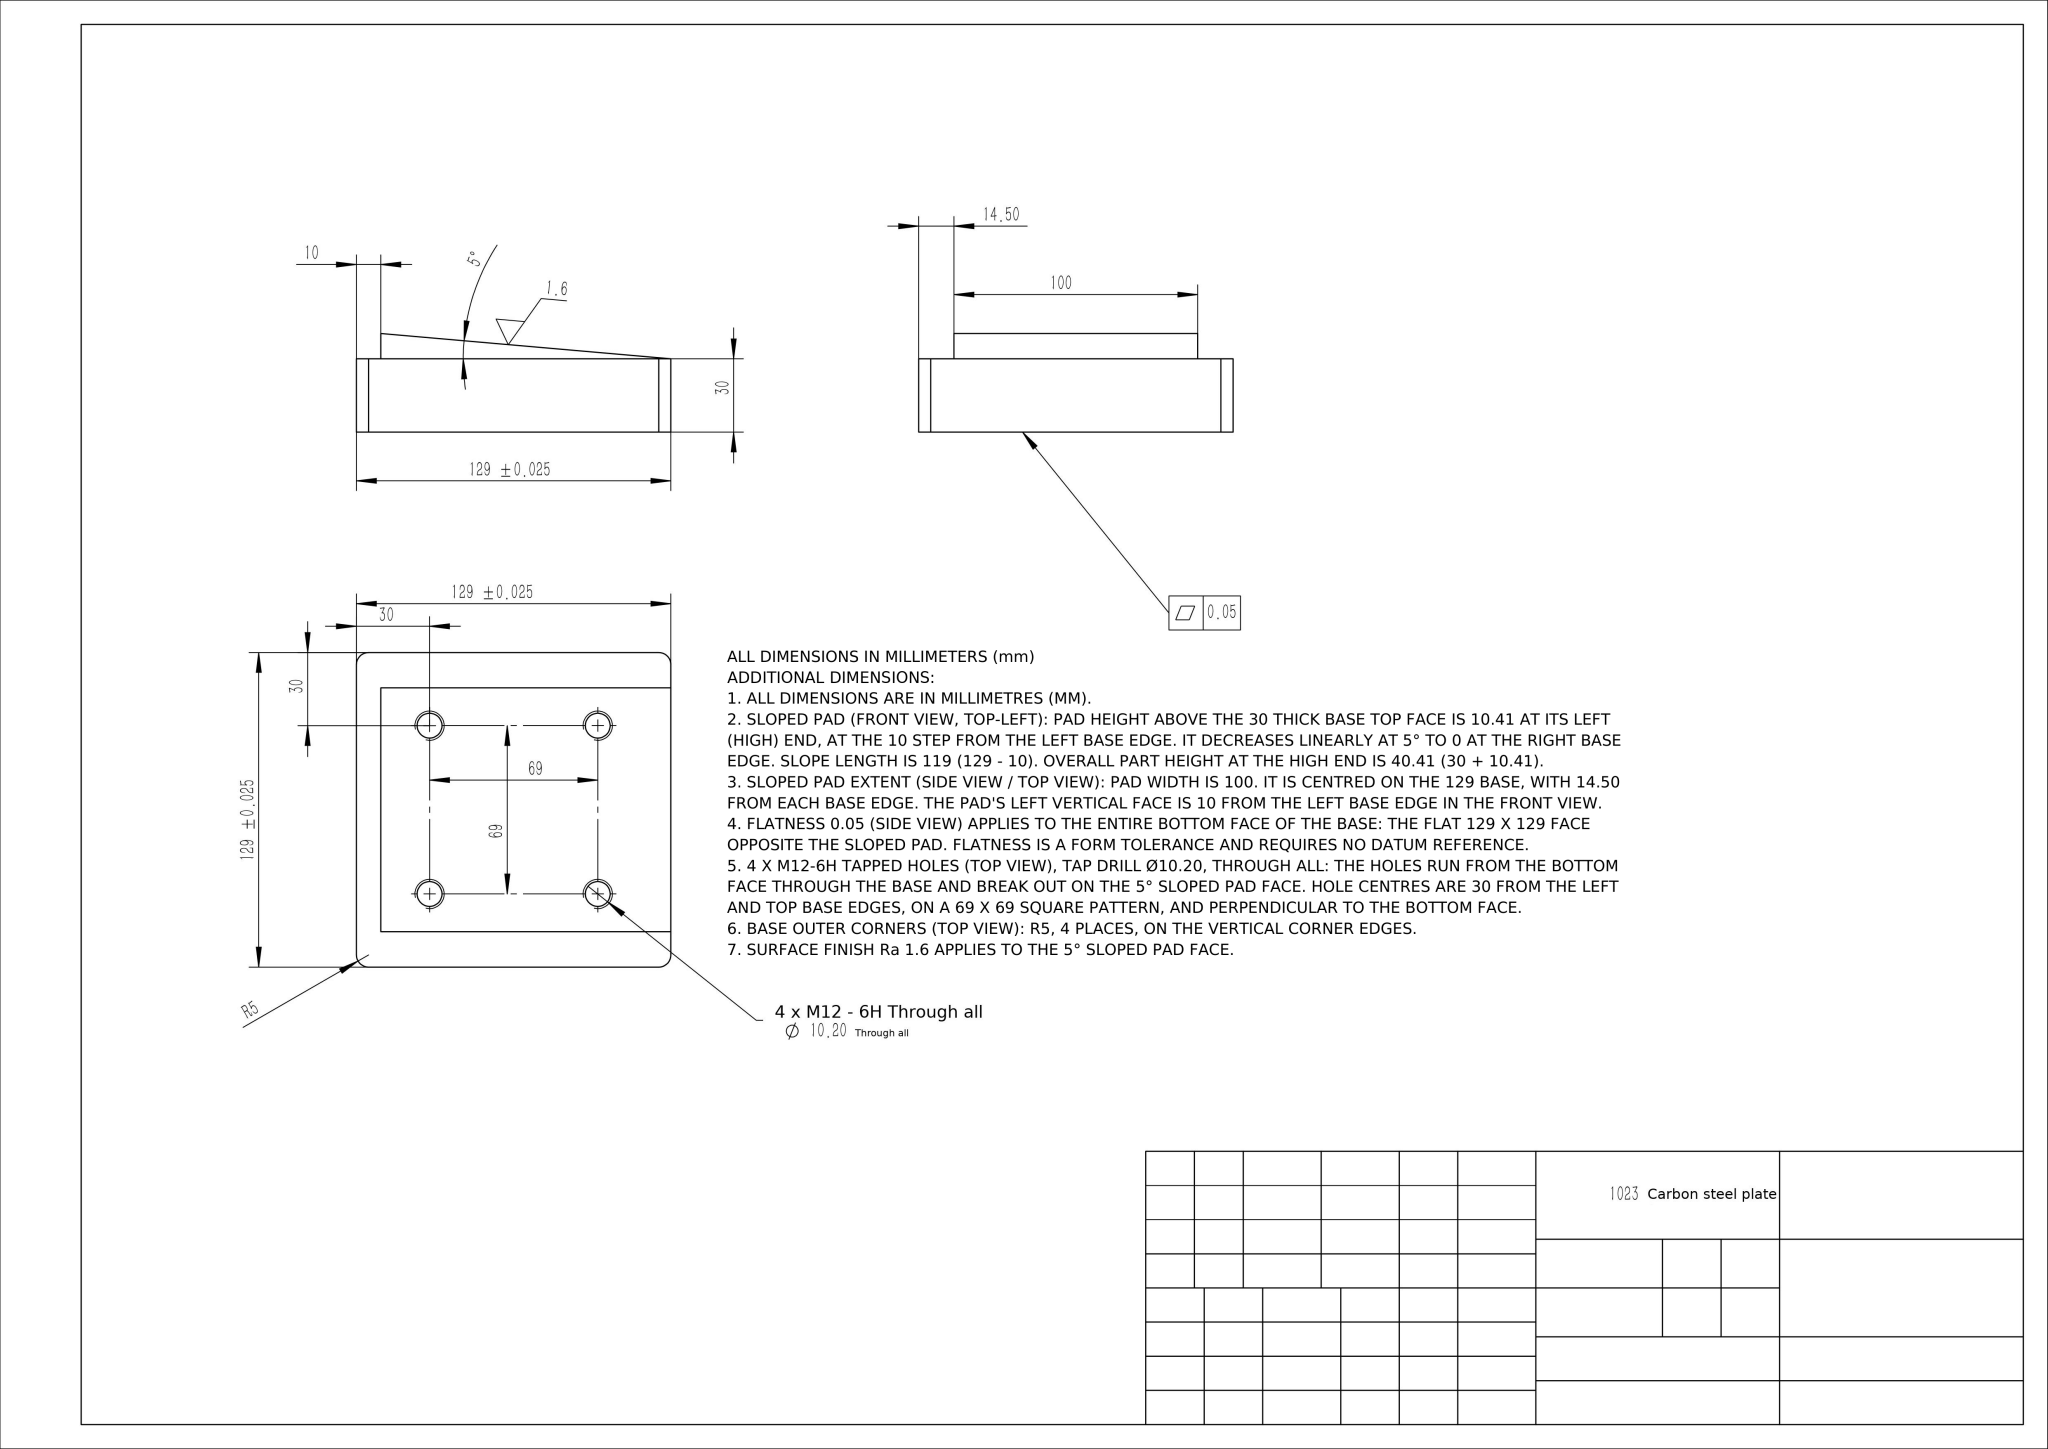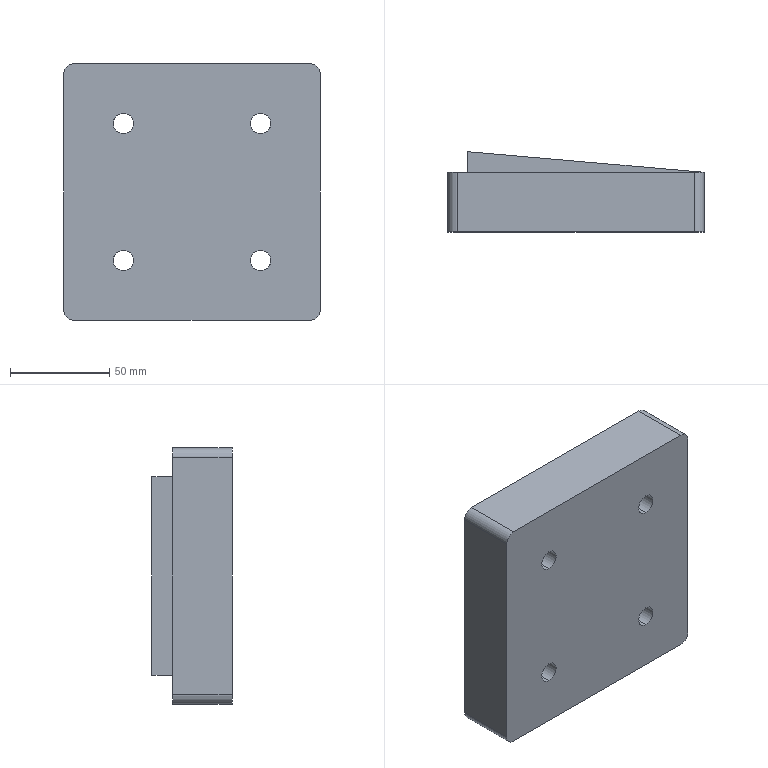Part | NX | mm | Chamfered Corner Four-Bore Rectangular Mounting Plate | 1 solid | 22 faces | box 129 x 40.41 x 129 mm | volume 548883 mm3 | cylinder 12 | plane 10 | commonest cylinder face diameters 10.2 x8 10 x4
STEP:
#1=CARTESIAN_POINT('',(20.,8.661,89.6));
#2=VERTEX_POINT('',#1);
#3=CARTESIAN_POINT('',(20.,8.661,79.4));
#4=VERTEX_POINT('',#3);
#5=CARTESIAN_POINT('',(20.,8.661,89.6));
#6=CARTESIAN_POINT('',(9.8,9.554,89.6));
#7=CARTESIAN_POINT('',(9.8,9.554,79.4));
#8=CARTESIAN_POINT('',(20.,8.661,79.4));
#9=(BOUNDED_CURVE()B_SPLINE_CURVE(3,(#5,#6,#7,#8),.UNSPECIFIED.,.F.,.F.)B_SPLINE_CURVE_WITH_KNOTS((4,4),(1.571,4.712),.UNSPECIFIED.)CURVE()GEOMETRIC_REPRESENTATION_ITEM()RATIONAL_B_SPLINE_CURVE((1.,0.3333,0.3333,1.))REPRESENTATION_ITEM(''));
#10=EDGE_CURVE('',#2,#4,#9,.T.);
#11=ORIENTED_EDGE('',*,*,#10,.F.);
#12=CARTESIAN_POINT('',(20.,-30.,89.6));
#13=VERTEX_POINT('',#12);
#14=CARTESIAN_POINT('',(20.,-30.,89.6));
#15=DIRECTION('',(0.,-1.,0.));
#16=VECTOR('',#15,1000.);
#17=LINE('',#14,#16);
#18=EDGE_CURVE('',#2,#13,#17,.T.);
#19=ORIENTED_EDGE('',*,*,#18,.T.);
#20=CARTESIAN_POINT('',(20.,-30.,79.4));
#21=VERTEX_POINT('',#20);
#22=CARTESIAN_POINT('',(20.,-30.,84.5));
#23=DIRECTION('',(0.,-1.,0.));
#24=DIRECTION('',(0.,0.,-1.));
#25=AXIS2_PLACEMENT_3D('',#22,#23,#24);
#26=CIRCLE('',#25,5.1);
#27=EDGE_CURVE('',#13,#21,#26,.T.);
#28=ORIENTED_EDGE('',*,*,#27,.T.);
#29=CARTESIAN_POINT('',(20.,-30.,79.4));
#30=DIRECTION('',(0.,-1.,0.));
#31=VECTOR('',#30,1000.);
#32=LINE('',#29,#31);
#33=EDGE_CURVE('',#4,#21,#32,.T.);
#34=ORIENTED_EDGE('',*,*,#33,.F.);
#35=EDGE_LOOP('',(#11,#19,#28,#34));
#36=FACE_OUTER_BOUND('',#35,.T.);
#37=CARTESIAN_POINT('',(20.,-30.,84.5));
#38=DIRECTION('',(0.,-1.,0.));
#39=DIRECTION('',(0.,0.,-1.));
#40=AXIS2_PLACEMENT_3D('',#37,#38,#39);
#41=CYLINDRICAL_SURFACE('',#40,5.1);
#42=ADVANCED_FACE('',(#36),#41,.F.);
#43=CARTESIAN_POINT('',(20.,8.661,20.6));
#44=VERTEX_POINT('',#43);
#45=CARTESIAN_POINT('',(20.,8.661,10.4));
#46=VERTEX_POINT('',#45);
#47=CARTESIAN_POINT('',(20.,8.661,20.6));
#48=CARTESIAN_POINT('',(9.8,9.554,20.6));
#49=CARTESIAN_POINT('',(9.8,9.554,10.4));
#50=CARTESIAN_POINT('',(20.,8.661,10.4));
#51=(BOUNDED_CURVE()B_SPLINE_CURVE(3,(#47,#48,#49,#50),.UNSPECIFIED.,.F.,.F.)B_SPLINE_CURVE_WITH_KNOTS((4,4),(1.571,4.712),.UNSPECIFIED.)CURVE()GEOMETRIC_REPRESENTATION_ITEM()RATIONAL_B_SPLINE_CURVE((1.,0.3333,0.3333,1.))REPRESENTATION_ITEM(''));
#52=EDGE_CURVE('',#44,#46,#51,.T.);
#53=ORIENTED_EDGE('',*,*,#52,.F.);
#54=CARTESIAN_POINT('',(20.,-30.,20.6));
#55=VERTEX_POINT('',#54);
#56=CARTESIAN_POINT('',(20.,-30.,20.6));
#57=DIRECTION('',(0.,-1.,0.));
#58=VECTOR('',#57,1000.);
#59=LINE('',#56,#58);
#60=EDGE_CURVE('',#44,#55,#59,.T.);
#61=ORIENTED_EDGE('',*,*,#60,.T.);
#62=CARTESIAN_POINT('',(20.,-30.,10.4));
#63=VERTEX_POINT('',#62);
#64=CARTESIAN_POINT('',(20.,-30.,15.5));
#65=DIRECTION('',(0.,-1.,0.));
#66=DIRECTION('',(0.,0.,-1.));
#67=AXIS2_PLACEMENT_3D('',#64,#65,#66);
#68=CIRCLE('',#67,5.1);
#69=EDGE_CURVE('',#55,#63,#68,.T.);
#70=ORIENTED_EDGE('',*,*,#69,.T.);
#71=CARTESIAN_POINT('',(20.,-30.,10.4));
#72=DIRECTION('',(0.,-1.,0.));
#73=VECTOR('',#72,1000.);
#74=LINE('',#71,#73);
#75=EDGE_CURVE('',#46,#63,#74,.T.);
#76=ORIENTED_EDGE('',*,*,#75,.F.);
#77=EDGE_LOOP('',(#53,#61,#70,#76));
#78=FACE_OUTER_BOUND('',#77,.T.);
#79=CARTESIAN_POINT('',(20.,-30.,15.5));
#80=DIRECTION('',(0.,-1.,0.));
#81=DIRECTION('',(0.,0.,-1.));
#82=AXIS2_PLACEMENT_3D('',#79,#80,#81);
#83=CYLINDRICAL_SURFACE('',#82,5.1);
#84=ADVANCED_FACE('',(#78),#83,.F.);
#85=CARTESIAN_POINT('',(89.,2.625,89.6));
#86=VERTEX_POINT('',#85);
#87=CARTESIAN_POINT('',(89.,2.625,79.4));
#88=VERTEX_POINT('',#87);
#89=CARTESIAN_POINT('',(89.,2.625,89.6));
#90=CARTESIAN_POINT('',(78.8,3.517,89.6));
#91=CARTESIAN_POINT('',(78.8,3.517,79.4));
#92=CARTESIAN_POINT('',(89.,2.625,79.4));
#93=(BOUNDED_CURVE()B_SPLINE_CURVE(3,(#89,#90,#91,#92),.UNSPECIFIED.,.F.,.F.)B_SPLINE_CURVE_WITH_KNOTS((4,4),(1.571,4.712),.UNSPECIFIED.)CURVE()GEOMETRIC_REPRESENTATION_ITEM()RATIONAL_B_SPLINE_CURVE((1.,0.3333,0.3333,1.))REPRESENTATION_ITEM(''));
#94=EDGE_CURVE('',#86,#88,#93,.T.);
#95=ORIENTED_EDGE('',*,*,#94,.F.);
#96=CARTESIAN_POINT('',(89.,-30.,89.6));
#97=VERTEX_POINT('',#96);
#98=CARTESIAN_POINT('',(89.,-30.,89.6));
#99=DIRECTION('',(0.,-1.,0.));
#100=VECTOR('',#99,1000.);
#101=LINE('',#98,#100);
#102=EDGE_CURVE('',#86,#97,#101,.T.);
#103=ORIENTED_EDGE('',*,*,#102,.T.);
#104=CARTESIAN_POINT('',(89.,-30.,79.4));
#105=VERTEX_POINT('',#104);
#106=CARTESIAN_POINT('',(89.,-30.,84.5));
#107=DIRECTION('',(0.,-1.,0.));
#108=DIRECTION('',(0.,0.,-1.));
#109=AXIS2_PLACEMENT_3D('',#106,#107,#108);
#110=CIRCLE('',#109,5.1);
#111=EDGE_CURVE('',#97,#105,#110,.T.);
#112=ORIENTED_EDGE('',*,*,#111,.T.);
#113=CARTESIAN_POINT('',(89.,-30.,79.4));
#114=DIRECTION('',(0.,-1.,0.));
#115=VECTOR('',#114,1000.);
#116=LINE('',#113,#115);
#117=EDGE_CURVE('',#88,#105,#116,.T.);
#118=ORIENTED_EDGE('',*,*,#117,.F.);
#119=EDGE_LOOP('',(#95,#103,#112,#118));
#120=FACE_OUTER_BOUND('',#119,.T.);
#121=CARTESIAN_POINT('',(89.,-30.,84.5));
#122=DIRECTION('',(0.,-1.,0.));
#123=DIRECTION('',(0.,0.,-1.));
#124=AXIS2_PLACEMENT_3D('',#121,#122,#123);
#125=CYLINDRICAL_SURFACE('',#124,5.1);
#126=ADVANCED_FACE('',(#120),#125,.F.);
#127=CARTESIAN_POINT('',(89.,2.625,20.6));
#128=VERTEX_POINT('',#127);
#129=CARTESIAN_POINT('',(89.,2.625,10.4));
#130=VERTEX_POINT('',#129);
#131=CARTESIAN_POINT('',(89.,2.625,20.6));
#132=CARTESIAN_POINT('',(78.8,3.517,20.6));
#133=CARTESIAN_POINT('',(78.8,3.517,10.4));
#134=CARTESIAN_POINT('',(89.,2.625,10.4));
#135=(BOUNDED_CURVE()B_SPLINE_CURVE(3,(#131,#132,#133,#134),.UNSPECIFIED.,.F.,.F.)B_SPLINE_CURVE_WITH_KNOTS((4,4),(1.571,4.712),.UNSPECIFIED.)CURVE()GEOMETRIC_REPRESENTATION_ITEM()RATIONAL_B_SPLINE_CURVE((1.,0.3333,0.3333,1.))REPRESENTATION_ITEM(''));
#136=EDGE_CURVE('',#128,#130,#135,.T.);
#137=ORIENTED_EDGE('',*,*,#136,.F.);
#138=CARTESIAN_POINT('',(89.,-30.,20.6));
#139=VERTEX_POINT('',#138);
#140=CARTESIAN_POINT('',(89.,-30.,20.6));
#141=DIRECTION('',(0.,-1.,0.));
#142=VECTOR('',#141,1000.);
#143=LINE('',#140,#142);
#144=EDGE_CURVE('',#128,#139,#143,.T.);
#145=ORIENTED_EDGE('',*,*,#144,.T.);
#146=CARTESIAN_POINT('',(89.,-30.,10.4));
#147=VERTEX_POINT('',#146);
#148=CARTESIAN_POINT('',(89.,-30.,15.5));
#149=DIRECTION('',(0.,-1.,0.));
#150=DIRECTION('',(0.,0.,-1.));
#151=AXIS2_PLACEMENT_3D('',#148,#149,#150);
#152=CIRCLE('',#151,5.1);
#153=EDGE_CURVE('',#139,#147,#152,.T.);
#154=ORIENTED_EDGE('',*,*,#153,.T.);
#155=CARTESIAN_POINT('',(89.,-30.,10.4));
#156=DIRECTION('',(0.,-1.,0.));
#157=VECTOR('',#156,1000.);
#158=LINE('',#155,#157);
#159=EDGE_CURVE('',#130,#147,#158,.T.);
#160=ORIENTED_EDGE('',*,*,#159,.F.);
#161=EDGE_LOOP('',(#137,#145,#154,#160));
#162=FACE_OUTER_BOUND('',#161,.T.);
#163=CARTESIAN_POINT('',(89.,-30.,15.5));
#164=DIRECTION('',(0.,-1.,0.));
#165=DIRECTION('',(0.,0.,-1.));
#166=AXIS2_PLACEMENT_3D('',#163,#164,#165);
#167=CYLINDRICAL_SURFACE('',#166,5.1);
#168=ADVANCED_FACE('',(#162),#167,.F.);
#169=CARTESIAN_POINT('',(20.,8.661,79.4));
#170=CARTESIAN_POINT('',(30.2,7.769,79.4));
#171=CARTESIAN_POINT('',(30.2,7.769,89.6));
#172=CARTESIAN_POINT('',(20.,8.661,89.6));
#173=(BOUNDED_CURVE()B_SPLINE_CURVE(3,(#169,#170,#171,#172),.UNSPECIFIED.,.F.,.F.)B_SPLINE_CURVE_WITH_KNOTS((4,4),(4.712,7.854),.UNSPECIFIED.)CURVE()GEOMETRIC_REPRESENTATION_ITEM()RATIONAL_B_SPLINE_CURVE((1.,0.3333,0.3333,1.))REPRESENTATION_ITEM(''));
#174=EDGE_CURVE('',#4,#2,#173,.T.);
#175=ORIENTED_EDGE('',*,*,#174,.T.);
#176=ORIENTED_EDGE('',*,*,#10,.T.);
#177=EDGE_LOOP('',(#175,#176));
#178=FACE_BOUND('',#177,.T.);
#179=CARTESIAN_POINT('',(20.,8.661,10.4));
#180=CARTESIAN_POINT('',(30.2,7.769,10.4));
#181=CARTESIAN_POINT('',(30.2,7.769,20.6));
#182=CARTESIAN_POINT('',(20.,8.661,20.6));
#183=(BOUNDED_CURVE()B_SPLINE_CURVE(3,(#179,#180,#181,#182),.UNSPECIFIED.,.F.,.F.)B_SPLINE_CURVE_WITH_KNOTS((4,4),(4.712,7.854),.UNSPECIFIED.)CURVE()GEOMETRIC_REPRESENTATION_ITEM()RATIONAL_B_SPLINE_CURVE((1.,0.3333,0.3333,1.))REPRESENTATION_ITEM(''));
#184=EDGE_CURVE('',#46,#44,#183,.T.);
#185=ORIENTED_EDGE('',*,*,#184,.T.);
#186=ORIENTED_EDGE('',*,*,#52,.T.);
#187=EDGE_LOOP('',(#185,#186));
#188=FACE_BOUND('',#187,.T.);
#189=CARTESIAN_POINT('',(89.,2.625,79.4));
#190=CARTESIAN_POINT('',(99.2,1.732,79.4));
#191=CARTESIAN_POINT('',(99.2,1.732,89.6));
#192=CARTESIAN_POINT('',(89.,2.625,89.6));
#193=(BOUNDED_CURVE()B_SPLINE_CURVE(3,(#189,#190,#191,#192),.UNSPECIFIED.,.F.,.F.)B_SPLINE_CURVE_WITH_KNOTS((4,4),(4.712,7.854),.UNSPECIFIED.)CURVE()GEOMETRIC_REPRESENTATION_ITEM()RATIONAL_B_SPLINE_CURVE((1.,0.3333,0.3333,1.))REPRESENTATION_ITEM(''));
#194=EDGE_CURVE('',#88,#86,#193,.T.);
#195=ORIENTED_EDGE('',*,*,#194,.T.);
#196=ORIENTED_EDGE('',*,*,#94,.T.);
#197=EDGE_LOOP('',(#195,#196));
#198=FACE_BOUND('',#197,.T.);
#199=CARTESIAN_POINT('',(89.,2.625,10.4));
#200=CARTESIAN_POINT('',(99.2,1.732,10.4));
#201=CARTESIAN_POINT('',(99.2,1.732,20.6));
#202=CARTESIAN_POINT('',(89.,2.625,20.6));
#203=(BOUNDED_CURVE()B_SPLINE_CURVE(3,(#199,#200,#201,#202),.UNSPECIFIED.,.F.,.F.)B_SPLINE_CURVE_WITH_KNOTS((4,4),(4.712,7.854),.UNSPECIFIED.)CURVE()GEOMETRIC_REPRESENTATION_ITEM()RATIONAL_B_SPLINE_CURVE((1.,0.3333,0.3333,1.))REPRESENTATION_ITEM(''));
#204=EDGE_CURVE('',#130,#128,#203,.T.);
#205=ORIENTED_EDGE('',*,*,#204,.T.);
#206=ORIENTED_EDGE('',*,*,#136,.T.);
#207=EDGE_LOOP('',(#205,#206));
#208=FACE_BOUND('',#207,.T.);
#209=CARTESIAN_POINT('',(119.,0.,0.));
#210=VERTEX_POINT('',#209);
#211=CARTESIAN_POINT('',(0.,10.411,0.));
#212=VERTEX_POINT('',#211);
#213=CARTESIAN_POINT('',(0.,10.411,0.));
#214=DIRECTION('',(-0.9962,0.08716,0.));
#215=VECTOR('',#214,1000.);
#216=LINE('',#213,#215);
#217=EDGE_CURVE('',#210,#212,#216,.T.);
#218=ORIENTED_EDGE('',*,*,#217,.T.);
#219=CARTESIAN_POINT('',(0.,10.411,100.));
#220=VERTEX_POINT('',#219);
#221=CARTESIAN_POINT('',(0.,10.411,100.));
#222=DIRECTION('',(0.,0.,-1.));
#223=VECTOR('',#222,1000.);
#224=LINE('',#221,#223);
#225=EDGE_CURVE('',#220,#212,#224,.T.);
#226=ORIENTED_EDGE('',*,*,#225,.F.);
#227=CARTESIAN_POINT('',(119.,0.,100.));
#228=VERTEX_POINT('',#227);
#229=CARTESIAN_POINT('',(0.,10.411,100.));
#230=DIRECTION('',(-0.9962,0.08716,0.));
#231=VECTOR('',#230,1000.);
#232=LINE('',#229,#231);
#233=EDGE_CURVE('',#228,#220,#232,.T.);
#234=ORIENTED_EDGE('',*,*,#233,.F.);
#235=CARTESIAN_POINT('',(119.,0.,100.));
#236=DIRECTION('',(0.,0.,-1.));
#237=VECTOR('',#236,1000.);
#238=LINE('',#235,#237);
#239=EDGE_CURVE('',#228,#210,#238,.T.);
#240=ORIENTED_EDGE('',*,*,#239,.T.);
#241=EDGE_LOOP('',(#218,#226,#234,#240));
#242=FACE_OUTER_BOUND('',#241,.T.);
#243=CARTESIAN_POINT('',(0.,10.411,100.));
#244=DIRECTION('',(-0.08716,-0.9962,0.));
#245=DIRECTION('',(0.9962,-0.08716,0.));
#246=AXIS2_PLACEMENT_3D('',#243,#244,#245);
#247=PLANE('',#246);
#248=ADVANCED_FACE('',(#178,#188,#198,#208,#242),#247,.F.);
#249=CARTESIAN_POINT('',(0.,0.,0.));
#250=VERTEX_POINT('',#249);
#251=CARTESIAN_POINT('',(0.,0.,0.));
#252=DIRECTION('',(-0.,-1.,0.));
#253=VECTOR('',#252,1000.);
#254=LINE('',#251,#253);
#255=EDGE_CURVE('',#212,#250,#254,.T.);
#256=ORIENTED_EDGE('',*,*,#255,.T.);
#257=CARTESIAN_POINT('',(0.,0.,100.));
#258=VERTEX_POINT('',#257);
#259=CARTESIAN_POINT('',(0.,0.,100.));
#260=DIRECTION('',(0.,0.,-1.));
#261=VECTOR('',#260,1000.);
#262=LINE('',#259,#261);
#263=EDGE_CURVE('',#258,#250,#262,.T.);
#264=ORIENTED_EDGE('',*,*,#263,.F.);
#265=CARTESIAN_POINT('',(0.,0.,100.));
#266=DIRECTION('',(-0.,-1.,0.));
#267=VECTOR('',#266,1000.);
#268=LINE('',#265,#267);
#269=EDGE_CURVE('',#220,#258,#268,.T.);
#270=ORIENTED_EDGE('',*,*,#269,.F.);
#271=ORIENTED_EDGE('',*,*,#225,.T.);
#272=EDGE_LOOP('',(#256,#264,#270,#271));
#273=FACE_OUTER_BOUND('',#272,.T.);
#274=CARTESIAN_POINT('',(0.,0.,100.));
#275=DIRECTION('',(1.,-0.,0.));
#276=DIRECTION('',(0.,1.,0.));
#277=AXIS2_PLACEMENT_3D('',#274,#275,#276);
#278=PLANE('',#277);
#279=ADVANCED_FACE('',(#273),#278,.F.);
#280=CARTESIAN_POINT('',(119.,0.,100.));
#281=DIRECTION('',(1.,0.,0.));
#282=VECTOR('',#281,1000.);
#283=LINE('',#280,#282);
#284=EDGE_CURVE('',#258,#228,#283,.T.);
#285=ORIENTED_EDGE('',*,*,#284,.T.);
#286=ORIENTED_EDGE('',*,*,#233,.T.);
#287=ORIENTED_EDGE('',*,*,#269,.T.);
#288=EDGE_LOOP('',(#285,#286,#287));
#289=FACE_OUTER_BOUND('',#288,.T.);
#290=CARTESIAN_POINT('',(0.,0.,100.));
#291=DIRECTION('',(0.,0.,-1.));
#292=DIRECTION('',(-1.,0.,0.));
#293=AXIS2_PLACEMENT_3D('',#290,#291,#292);
#294=PLANE('',#293);
#295=ADVANCED_FACE('',(#289),#294,.F.);
#296=CARTESIAN_POINT('',(119.,0.,0.));
#297=DIRECTION('',(1.,0.,0.));
#298=VECTOR('',#297,1000.);
#299=LINE('',#296,#298);
#300=EDGE_CURVE('',#250,#210,#299,.T.);
#301=ORIENTED_EDGE('',*,*,#300,.F.);
#302=ORIENTED_EDGE('',*,*,#255,.F.);
#303=ORIENTED_EDGE('',*,*,#217,.F.);
#304=EDGE_LOOP('',(#301,#302,#303));
#305=FACE_OUTER_BOUND('',#304,.T.);
#306=CARTESIAN_POINT('',(0.,0.,0.));
#307=DIRECTION('',(0.,0.,-1.));
#308=DIRECTION('',(-1.,0.,0.));
#309=AXIS2_PLACEMENT_3D('',#306,#307,#308);
#310=PLANE('',#309);
#311=ADVANCED_FACE('',(#305),#310,.T.);
#312=CARTESIAN_POINT('',(-10.,-0.,109.5));
#313=VERTEX_POINT('',#312);
#314=CARTESIAN_POINT('',(-10.,-0.,-9.5));
#315=VERTEX_POINT('',#314);
#316=CARTESIAN_POINT('',(-10.,-0.,114.5));
#317=DIRECTION('',(0.,0.,-1.));
#318=VECTOR('',#317,1000.);
#319=LINE('',#316,#318);
#320=EDGE_CURVE('',#313,#315,#319,.T.);
#321=ORIENTED_EDGE('',*,*,#320,.F.);
#322=CARTESIAN_POINT('',(-5.,-0.,114.5));
#323=VERTEX_POINT('',#322);
#324=CARTESIAN_POINT('',(-5.,0.,109.5));
#325=DIRECTION('',(-0.,1.,0.));
#326=DIRECTION('',(1.,0.,0.));
#327=AXIS2_PLACEMENT_3D('',#324,#325,#326);
#328=CIRCLE('',#327,5.);
#329=EDGE_CURVE('',#313,#323,#328,.T.);
#330=ORIENTED_EDGE('',*,*,#329,.T.);
#331=CARTESIAN_POINT('',(114.,0.,114.5));
#332=VERTEX_POINT('',#331);
#333=CARTESIAN_POINT('',(-10.,-0.,114.5));
#334=DIRECTION('',(-1.,-0.,0.));
#335=VECTOR('',#334,1000.);
#336=LINE('',#333,#335);
#337=EDGE_CURVE('',#332,#323,#336,.T.);
#338=ORIENTED_EDGE('',*,*,#337,.F.);
#339=CARTESIAN_POINT('',(119.,0.,109.5));
#340=VERTEX_POINT('',#339);
#341=CARTESIAN_POINT('',(114.,0.,109.5));
#342=DIRECTION('',(-0.,1.,0.));
#343=DIRECTION('',(1.,0.,0.));
#344=AXIS2_PLACEMENT_3D('',#341,#342,#343);
#345=CIRCLE('',#344,5.);
#346=EDGE_CURVE('',#332,#340,#345,.T.);
#347=ORIENTED_EDGE('',*,*,#346,.T.);
#348=CARTESIAN_POINT('',(119.,0.,114.5));
#349=DIRECTION('',(-0.,-0.,1.));
#350=VECTOR('',#349,1000.);
#351=LINE('',#348,#350);
#352=EDGE_CURVE('',#228,#340,#351,.T.);
#353=ORIENTED_EDGE('',*,*,#352,.F.);
#354=ORIENTED_EDGE('',*,*,#284,.F.);
#355=ORIENTED_EDGE('',*,*,#263,.T.);
#356=ORIENTED_EDGE('',*,*,#300,.T.);
#357=CARTESIAN_POINT('',(119.,0.,-9.5));
#358=VERTEX_POINT('',#357);
#359=CARTESIAN_POINT('',(119.,0.,114.5));
#360=DIRECTION('',(-0.,-0.,1.));
#361=VECTOR('',#360,1000.);
#362=LINE('',#359,#361);
#363=EDGE_CURVE('',#358,#210,#362,.T.);
#364=ORIENTED_EDGE('',*,*,#363,.F.);
#365=CARTESIAN_POINT('',(114.,0.,-14.5));
#366=VERTEX_POINT('',#365);
#367=CARTESIAN_POINT('',(114.,0.,-9.5));
#368=DIRECTION('',(-0.,1.,0.));
#369=DIRECTION('',(1.,0.,0.));
#370=AXIS2_PLACEMENT_3D('',#367,#368,#369);
#371=CIRCLE('',#370,5.);
#372=EDGE_CURVE('',#358,#366,#371,.T.);
#373=ORIENTED_EDGE('',*,*,#372,.T.);
#374=CARTESIAN_POINT('',(-5.,-0.,-14.5));
#375=VERTEX_POINT('',#374);
#376=CARTESIAN_POINT('',(-10.,-0.,-14.5));
#377=DIRECTION('',(1.,0.,0.));
#378=VECTOR('',#377,1000.);
#379=LINE('',#376,#378);
#380=EDGE_CURVE('',#375,#366,#379,.T.);
#381=ORIENTED_EDGE('',*,*,#380,.F.);
#382=CARTESIAN_POINT('',(-5.,0.,-9.5));
#383=DIRECTION('',(-0.,1.,0.));
#384=DIRECTION('',(1.,0.,0.));
#385=AXIS2_PLACEMENT_3D('',#382,#383,#384);
#386=CIRCLE('',#385,5.);
#387=EDGE_CURVE('',#375,#315,#386,.T.);
#388=ORIENTED_EDGE('',*,*,#387,.T.);
#389=EDGE_LOOP('',(#321,#330,#338,#347,#353,#354,#355,#356,#364,#373,#381,#388));
#390=FACE_OUTER_BOUND('',#389,.T.);
#391=CARTESIAN_POINT('',(0.,-0.,-0.));
#392=DIRECTION('',(0.,-1.,-0.));
#393=DIRECTION('',(1.,0.,0.));
#394=AXIS2_PLACEMENT_3D('',#391,#392,#393);
#395=PLANE('',#394);
#396=ADVANCED_FACE('',(#390),#395,.F.);
#397=CARTESIAN_POINT('',(119.,-30.,-9.5));
#398=VERTEX_POINT('',#397);
#399=CARTESIAN_POINT('',(119.,-30.,109.5));
#400=VERTEX_POINT('',#399);
#401=CARTESIAN_POINT('',(119.,-30.,114.5));
#402=DIRECTION('',(-0.,-0.,1.));
#403=VECTOR('',#402,1000.);
#404=LINE('',#401,#403);
#405=EDGE_CURVE('',#398,#400,#404,.T.);
#406=ORIENTED_EDGE('',*,*,#405,.F.);
#407=CARTESIAN_POINT('',(119.,-30.,-9.5));
#408=DIRECTION('',(-0.,1.,0.));
#409=VECTOR('',#408,1000.);
#410=LINE('',#407,#409);
#411=EDGE_CURVE('',#398,#358,#410,.T.);
#412=ORIENTED_EDGE('',*,*,#411,.T.);
#413=ORIENTED_EDGE('',*,*,#363,.T.);
#414=ORIENTED_EDGE('',*,*,#239,.F.);
#415=ORIENTED_EDGE('',*,*,#352,.T.);
#416=CARTESIAN_POINT('',(119.,-30.,109.5));
#417=DIRECTION('',(0.,-1.,0.));
#418=VECTOR('',#417,1000.);
#419=LINE('',#416,#418);
#420=EDGE_CURVE('',#340,#400,#419,.T.);
#421=ORIENTED_EDGE('',*,*,#420,.T.);
#422=EDGE_LOOP('',(#406,#412,#413,#414,#415,#421));
#423=FACE_OUTER_BOUND('',#422,.T.);
#424=CARTESIAN_POINT('',(119.,-30.,114.5));
#425=DIRECTION('',(-1.,-0.,-0.));
#426=DIRECTION('',(-0.,0.,1.));
#427=AXIS2_PLACEMENT_3D('',#424,#425,#426);
#428=PLANE('',#427);
#429=ADVANCED_FACE('',(#423),#428,.F.);
#430=ORIENTED_EDGE('',*,*,#337,.T.);
#431=CARTESIAN_POINT('',(-5.,-30.,114.5));
#432=VERTEX_POINT('',#431);
#433=CARTESIAN_POINT('',(-5.,-30.,114.5));
#434=DIRECTION('',(0.,-1.,0.));
#435=VECTOR('',#434,1000.);
#436=LINE('',#433,#435);
#437=EDGE_CURVE('',#323,#432,#436,.T.);
#438=ORIENTED_EDGE('',*,*,#437,.T.);
#439=CARTESIAN_POINT('',(114.,-30.,114.5));
#440=VERTEX_POINT('',#439);
#441=CARTESIAN_POINT('',(-10.,-30.,114.5));
#442=DIRECTION('',(-1.,-0.,0.));
#443=VECTOR('',#442,1000.);
#444=LINE('',#441,#443);
#445=EDGE_CURVE('',#440,#432,#444,.T.);
#446=ORIENTED_EDGE('',*,*,#445,.F.);
#447=CARTESIAN_POINT('',(114.,-30.,114.5));
#448=DIRECTION('',(-0.,1.,0.));
#449=VECTOR('',#448,1000.);
#450=LINE('',#447,#449);
#451=EDGE_CURVE('',#440,#332,#450,.T.);
#452=ORIENTED_EDGE('',*,*,#451,.T.);
#453=EDGE_LOOP('',(#430,#438,#446,#452));
#454=FACE_OUTER_BOUND('',#453,.T.);
#455=CARTESIAN_POINT('',(-10.,-30.,114.5));
#456=DIRECTION('',(0.,0.,-1.));
#457=DIRECTION('',(-1.,0.,0.));
#458=AXIS2_PLACEMENT_3D('',#455,#456,#457);
#459=PLANE('',#458);
#460=ADVANCED_FACE('',(#454),#459,.F.);
#461=CARTESIAN_POINT('',(-10.,-30.,109.5));
#462=VERTEX_POINT('',#461);
#463=CARTESIAN_POINT('',(-10.,-30.,-9.5));
#464=VERTEX_POINT('',#463);
#465=CARTESIAN_POINT('',(-10.,-30.,114.5));
#466=DIRECTION('',(0.,0.,-1.));
#467=VECTOR('',#466,1000.);
#468=LINE('',#465,#467);
#469=EDGE_CURVE('',#462,#464,#468,.T.);
#470=ORIENTED_EDGE('',*,*,#469,.F.);
#471=CARTESIAN_POINT('',(-10.,-30.,109.5));
#472=DIRECTION('',(-0.,1.,0.));
#473=VECTOR('',#472,1000.);
#474=LINE('',#471,#473);
#475=EDGE_CURVE('',#462,#313,#474,.T.);
#476=ORIENTED_EDGE('',*,*,#475,.T.);
#477=ORIENTED_EDGE('',*,*,#320,.T.);
#478=CARTESIAN_POINT('',(-10.,-30.,-9.5));
#479=DIRECTION('',(0.,-1.,0.));
#480=VECTOR('',#479,1000.);
#481=LINE('',#478,#480);
#482=EDGE_CURVE('',#315,#464,#481,.T.);
#483=ORIENTED_EDGE('',*,*,#482,.T.);
#484=EDGE_LOOP('',(#470,#476,#477,#483));
#485=FACE_OUTER_BOUND('',#484,.T.);
#486=CARTESIAN_POINT('',(-10.,-30.,114.5));
#487=DIRECTION('',(1.,0.,0.));
#488=DIRECTION('',(0.,0.,-1.));
#489=AXIS2_PLACEMENT_3D('',#486,#487,#488);
#490=PLANE('',#489);
#491=ADVANCED_FACE('',(#485),#490,.F.);
#492=CARTESIAN_POINT('',(-5.,-30.,-14.5));
#493=VERTEX_POINT('',#492);
#494=CARTESIAN_POINT('',(114.,-30.,-14.5));
#495=VERTEX_POINT('',#494);
#496=CARTESIAN_POINT('',(-10.,-30.,-14.5));
#497=DIRECTION('',(1.,0.,0.));
#498=VECTOR('',#497,1000.);
#499=LINE('',#496,#498);
#500=EDGE_CURVE('',#493,#495,#499,.T.);
#501=ORIENTED_EDGE('',*,*,#500,.F.);
#502=CARTESIAN_POINT('',(-5.,-30.,-14.5));
#503=DIRECTION('',(-0.,1.,0.));
#504=VECTOR('',#503,1000.);
#505=LINE('',#502,#504);
#506=EDGE_CURVE('',#493,#375,#505,.T.);
#507=ORIENTED_EDGE('',*,*,#506,.T.);
#508=ORIENTED_EDGE('',*,*,#380,.T.);
#509=CARTESIAN_POINT('',(114.,-30.,-14.5));
#510=DIRECTION('',(0.,-1.,0.));
#511=VECTOR('',#510,1000.);
#512=LINE('',#509,#511);
#513=EDGE_CURVE('',#366,#495,#512,.T.);
#514=ORIENTED_EDGE('',*,*,#513,.T.);
#515=EDGE_LOOP('',(#501,#507,#508,#514));
#516=FACE_OUTER_BOUND('',#515,.T.);
#517=CARTESIAN_POINT('',(-10.,-30.,-14.5));
#518=DIRECTION('',(0.,0.,1.));
#519=DIRECTION('',(1.,0.,0.));
#520=AXIS2_PLACEMENT_3D('',#517,#518,#519);
#521=PLANE('',#520);
#522=ADVANCED_FACE('',(#516),#521,.F.);
#523=CARTESIAN_POINT('',(20.,-30.,84.5));
#524=DIRECTION('',(0.,-1.,0.));
#525=DIRECTION('',(0.,0.,-1.));
#526=AXIS2_PLACEMENT_3D('',#523,#524,#525);
#527=CIRCLE('',#526,5.1);
#528=EDGE_CURVE('',#21,#13,#527,.T.);
#529=ORIENTED_EDGE('',*,*,#528,.F.);
#530=ORIENTED_EDGE('',*,*,#27,.F.);
#531=EDGE_LOOP('',(#529,#530));
#532=FACE_BOUND('',#531,.T.);
#533=CARTESIAN_POINT('',(20.,-30.,15.5));
#534=DIRECTION('',(0.,-1.,0.));
#535=DIRECTION('',(0.,0.,-1.));
#536=AXIS2_PLACEMENT_3D('',#533,#534,#535);
#537=CIRCLE('',#536,5.1);
#538=EDGE_CURVE('',#63,#55,#537,.T.);
#539=ORIENTED_EDGE('',*,*,#538,.F.);
#540=ORIENTED_EDGE('',*,*,#69,.F.);
#541=EDGE_LOOP('',(#539,#540));
#542=FACE_BOUND('',#541,.T.);
#543=CARTESIAN_POINT('',(89.,-30.,84.5));
#544=DIRECTION('',(0.,-1.,0.));
#545=DIRECTION('',(0.,0.,-1.));
#546=AXIS2_PLACEMENT_3D('',#543,#544,#545);
#547=CIRCLE('',#546,5.1);
#548=EDGE_CURVE('',#105,#97,#547,.T.);
#549=ORIENTED_EDGE('',*,*,#548,.F.);
#550=ORIENTED_EDGE('',*,*,#111,.F.);
#551=EDGE_LOOP('',(#549,#550));
#552=FACE_BOUND('',#551,.T.);
#553=CARTESIAN_POINT('',(89.,-30.,15.5));
#554=DIRECTION('',(0.,-1.,0.));
#555=DIRECTION('',(0.,0.,-1.));
#556=AXIS2_PLACEMENT_3D('',#553,#554,#555);
#557=CIRCLE('',#556,5.1);
#558=EDGE_CURVE('',#147,#139,#557,.T.);
#559=ORIENTED_EDGE('',*,*,#558,.F.);
#560=ORIENTED_EDGE('',*,*,#153,.F.);
#561=EDGE_LOOP('',(#559,#560));
#562=FACE_BOUND('',#561,.T.);
#563=ORIENTED_EDGE('',*,*,#445,.T.);
#564=CARTESIAN_POINT('',(-5.,-30.,109.5));
#565=DIRECTION('',(0.,-1.,-0.));
#566=DIRECTION('',(1.,0.,0.));
#567=AXIS2_PLACEMENT_3D('',#564,#565,#566);
#568=CIRCLE('',#567,5.);
#569=EDGE_CURVE('',#432,#462,#568,.T.);
#570=ORIENTED_EDGE('',*,*,#569,.T.);
#571=ORIENTED_EDGE('',*,*,#469,.T.);
#572=CARTESIAN_POINT('',(-5.,-30.,-9.5));
#573=DIRECTION('',(0.,-1.,-0.));
#574=DIRECTION('',(1.,0.,0.));
#575=AXIS2_PLACEMENT_3D('',#572,#573,#574);
#576=CIRCLE('',#575,5.);
#577=EDGE_CURVE('',#464,#493,#576,.T.);
#578=ORIENTED_EDGE('',*,*,#577,.T.);
#579=ORIENTED_EDGE('',*,*,#500,.T.);
#580=CARTESIAN_POINT('',(114.,-30.,-9.5));
#581=DIRECTION('',(0.,-1.,-0.));
#582=DIRECTION('',(1.,0.,0.));
#583=AXIS2_PLACEMENT_3D('',#580,#581,#582);
#584=CIRCLE('',#583,5.);
#585=EDGE_CURVE('',#495,#398,#584,.T.);
#586=ORIENTED_EDGE('',*,*,#585,.T.);
#587=ORIENTED_EDGE('',*,*,#405,.T.);
#588=CARTESIAN_POINT('',(114.,-30.,109.5));
#589=DIRECTION('',(0.,-1.,-0.));
#590=DIRECTION('',(1.,0.,0.));
#591=AXIS2_PLACEMENT_3D('',#588,#589,#590);
#592=CIRCLE('',#591,5.);
#593=EDGE_CURVE('',#400,#440,#592,.T.);
#594=ORIENTED_EDGE('',*,*,#593,.T.);
#595=EDGE_LOOP('',(#563,#570,#571,#578,#579,#586,#587,#594));
#596=FACE_OUTER_BOUND('',#595,.T.);
#597=CARTESIAN_POINT('',(0.,-30.,-0.));
#598=DIRECTION('',(0.,-1.,-0.));
#599=DIRECTION('',(1.,0.,0.));
#600=AXIS2_PLACEMENT_3D('',#597,#598,#599);
#601=PLANE('',#600);
#602=ADVANCED_FACE('',(#532,#542,#552,#562,#596),#601,.T.);
#603=ORIENTED_EDGE('',*,*,#144,.F.);
#604=ORIENTED_EDGE('',*,*,#204,.F.);
#605=ORIENTED_EDGE('',*,*,#159,.T.);
#606=ORIENTED_EDGE('',*,*,#558,.T.);
#607=EDGE_LOOP('',(#603,#604,#605,#606));
#608=FACE_OUTER_BOUND('',#607,.T.);
#609=CARTESIAN_POINT('',(89.,-30.,15.5));
#610=DIRECTION('',(0.,-1.,0.));
#611=DIRECTION('',(0.,0.,-1.));
#612=AXIS2_PLACEMENT_3D('',#609,#610,#611);
#613=CYLINDRICAL_SURFACE('',#612,5.1);
#614=ADVANCED_FACE('',(#608),#613,.F.);
#615=ORIENTED_EDGE('',*,*,#102,.F.);
#616=ORIENTED_EDGE('',*,*,#194,.F.);
#617=ORIENTED_EDGE('',*,*,#117,.T.);
#618=ORIENTED_EDGE('',*,*,#548,.T.);
#619=EDGE_LOOP('',(#615,#616,#617,#618));
#620=FACE_OUTER_BOUND('',#619,.T.);
#621=CARTESIAN_POINT('',(89.,-30.,84.5));
#622=DIRECTION('',(0.,-1.,0.));
#623=DIRECTION('',(0.,0.,-1.));
#624=AXIS2_PLACEMENT_3D('',#621,#622,#623);
#625=CYLINDRICAL_SURFACE('',#624,5.1);
#626=ADVANCED_FACE('',(#620),#625,.F.);
#627=ORIENTED_EDGE('',*,*,#60,.F.);
#628=ORIENTED_EDGE('',*,*,#184,.F.);
#629=ORIENTED_EDGE('',*,*,#75,.T.);
#630=ORIENTED_EDGE('',*,*,#538,.T.);
#631=EDGE_LOOP('',(#627,#628,#629,#630));
#632=FACE_OUTER_BOUND('',#631,.T.);
#633=CARTESIAN_POINT('',(20.,-30.,15.5));
#634=DIRECTION('',(0.,-1.,0.));
#635=DIRECTION('',(0.,0.,-1.));
#636=AXIS2_PLACEMENT_3D('',#633,#634,#635);
#637=CYLINDRICAL_SURFACE('',#636,5.1);
#638=ADVANCED_FACE('',(#632),#637,.F.);
#639=ORIENTED_EDGE('',*,*,#18,.F.);
#640=ORIENTED_EDGE('',*,*,#174,.F.);
#641=ORIENTED_EDGE('',*,*,#33,.T.);
#642=ORIENTED_EDGE('',*,*,#528,.T.);
#643=EDGE_LOOP('',(#639,#640,#641,#642));
#644=FACE_OUTER_BOUND('',#643,.T.);
#645=CARTESIAN_POINT('',(20.,-30.,84.5));
#646=DIRECTION('',(0.,-1.,0.));
#647=DIRECTION('',(0.,0.,-1.));
#648=AXIS2_PLACEMENT_3D('',#645,#646,#647);
#649=CYLINDRICAL_SURFACE('',#648,5.1);
#650=ADVANCED_FACE('',(#644),#649,.F.);
#651=ORIENTED_EDGE('',*,*,#569,.F.);
#652=ORIENTED_EDGE('',*,*,#437,.F.);
#653=ORIENTED_EDGE('',*,*,#329,.F.);
#654=ORIENTED_EDGE('',*,*,#475,.F.);
#655=EDGE_LOOP('',(#651,#652,#653,#654));
#656=FACE_OUTER_BOUND('',#655,.T.);
#657=CARTESIAN_POINT('',(-5.,-30.,109.5));
#658=DIRECTION('',(-0.,1.,0.));
#659=DIRECTION('',(-1.,0.,0.));
#660=AXIS2_PLACEMENT_3D('',#657,#658,#659);
#661=CYLINDRICAL_SURFACE('',#660,5.);
#662=ADVANCED_FACE('',(#656),#661,.T.);
#663=ORIENTED_EDGE('',*,*,#577,.F.);
#664=ORIENTED_EDGE('',*,*,#482,.F.);
#665=ORIENTED_EDGE('',*,*,#387,.F.);
#666=ORIENTED_EDGE('',*,*,#506,.F.);
#667=EDGE_LOOP('',(#663,#664,#665,#666));
#668=FACE_OUTER_BOUND('',#667,.T.);
#669=CARTESIAN_POINT('',(-5.,-30.,-9.5));
#670=DIRECTION('',(-0.,1.,0.));
#671=DIRECTION('',(-1.,0.,0.));
#672=AXIS2_PLACEMENT_3D('',#669,#670,#671);
#673=CYLINDRICAL_SURFACE('',#672,5.);
#674=ADVANCED_FACE('',(#668),#673,.T.);
#675=ORIENTED_EDGE('',*,*,#585,.F.);
#676=ORIENTED_EDGE('',*,*,#513,.F.);
#677=ORIENTED_EDGE('',*,*,#372,.F.);
#678=ORIENTED_EDGE('',*,*,#411,.F.);
#679=EDGE_LOOP('',(#675,#676,#677,#678));
#680=FACE_OUTER_BOUND('',#679,.T.);
#681=CARTESIAN_POINT('',(114.,-30.,-9.5));
#682=DIRECTION('',(-0.,1.,0.));
#683=DIRECTION('',(-1.,0.,0.));
#684=AXIS2_PLACEMENT_3D('',#681,#682,#683);
#685=CYLINDRICAL_SURFACE('',#684,5.);
#686=ADVANCED_FACE('',(#680),#685,.T.);
#687=ORIENTED_EDGE('',*,*,#593,.F.);
#688=ORIENTED_EDGE('',*,*,#420,.F.);
#689=ORIENTED_EDGE('',*,*,#346,.F.);
#690=ORIENTED_EDGE('',*,*,#451,.F.);
#691=EDGE_LOOP('',(#687,#688,#689,#690));
#692=FACE_OUTER_BOUND('',#691,.T.);
#693=CARTESIAN_POINT('',(114.,-30.,109.5));
#694=DIRECTION('',(-0.,1.,0.));
#695=DIRECTION('',(-1.,0.,0.));
#696=AXIS2_PLACEMENT_3D('',#693,#694,#695);
#697=CYLINDRICAL_SURFACE('',#696,5.);
#698=ADVANCED_FACE('',(#692),#697,.T.);
#699=CLOSED_SHELL('',(#42,#84,#126,#168,#248,#279,#295,#311,#396,#429,#460,#491,#522,#602,#614,#626,#638,#650,#662,#674,#686,#698));
#700=MANIFOLD_SOLID_BREP('',#699);
#701=CARTESIAN_POINT('',(0.,0.,0.));
#702=DIRECTION('',(0.,0.,1.));
#703=DIRECTION('',(1.,0.,0.));
#704=AXIS2_PLACEMENT_3D('',#701,#702,#703);
#705=(LENGTH_UNIT()NAMED_UNIT(*)SI_UNIT(.MILLI.,.METRE.));
#706=UNCERTAINTY_MEASURE_WITH_UNIT(LENGTH_MEASURE(0.00001),#705,'','');
#707=(NAMED_UNIT(*)PLANE_ANGLE_UNIT()SI_UNIT($,.RADIAN.));
#708=(NAMED_UNIT(*)SI_UNIT($,.STERADIAN.)SOLID_ANGLE_UNIT());
#709=(GEOMETRIC_REPRESENTATION_CONTEXT(3)GLOBAL_UNCERTAINTY_ASSIGNED_CONTEXT((#706))GLOBAL_UNIT_ASSIGNED_CONTEXT((#705,#707,#708))REPRESENTATION_CONTEXT('',''));
#710=ADVANCED_BREP_SHAPE_REPRESENTATION('',(#700,#704),#709);
#711=COLOUR_RGB('',0.7922,0.8196,0.9333);
#712=FILL_AREA_STYLE_COLOUR('',#711);
#713=FILL_AREA_STYLE('',(#712));
#714=SURFACE_STYLE_FILL_AREA(#713);
#715=SURFACE_SIDE_STYLE('',(#714));
#716=SURFACE_STYLE_USAGE(.BOTH.,#715);
#717=PRESENTATION_STYLE_ASSIGNMENT((#716));
#718=STYLED_ITEM('',(#717),#700);
#719=(LENGTH_UNIT()NAMED_UNIT(*)SI_UNIT(.MILLI.,.METRE.));
#720=UNCERTAINTY_MEASURE_WITH_UNIT(LENGTH_MEASURE(0.00001),#719,'','');
#721=(NAMED_UNIT(*)PLANE_ANGLE_UNIT()SI_UNIT($,.RADIAN.));
#722=(NAMED_UNIT(*)SI_UNIT($,.STERADIAN.)SOLID_ANGLE_UNIT());
#723=(GEOMETRIC_REPRESENTATION_CONTEXT(3)GLOBAL_UNCERTAINTY_ASSIGNED_CONTEXT((#720))GLOBAL_UNIT_ASSIGNED_CONTEXT((#719,#721,#722))REPRESENTATION_CONTEXT('',''));
#724=MECHANICAL_DESIGN_GEOMETRIC_PRESENTATION_REPRESENTATION('',(#718),#723);
#725=PRESENTATION_LAYER_ASSIGNMENT('','',(#718));